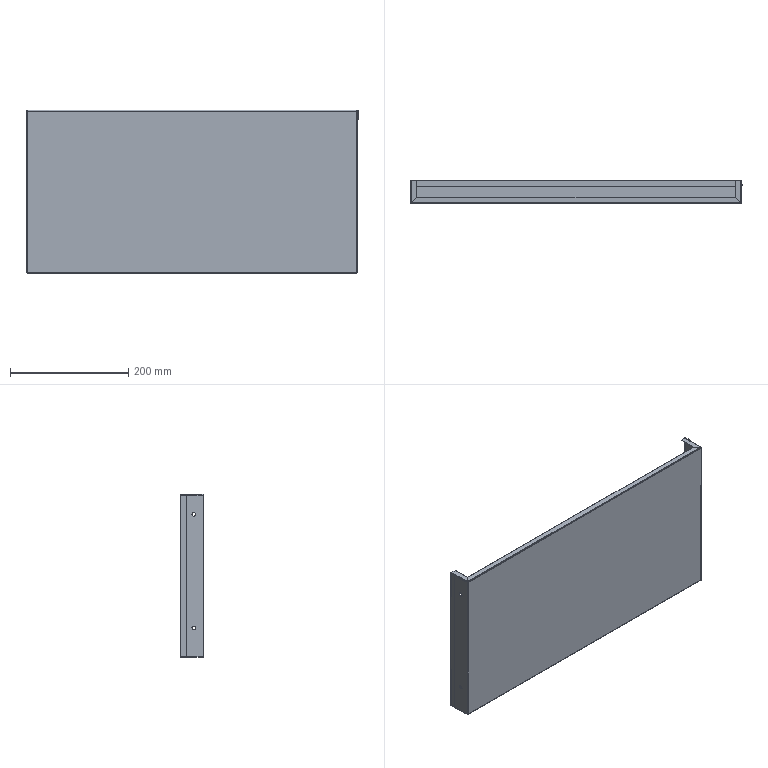Component | SolidWorks | PC-CAJ-P09-1_PC-CAJ-P14-1_PM-CAJ-P36-1 | 1 solid | 95 faces | volume 149083 mm3 | plane 62 | cylinder 29 | spline 4 | commonest cylinder face diameters 6 x8 1 x6 2.4 x6 1.6 x5 0.2 x4 | material Plain Carbon Steel